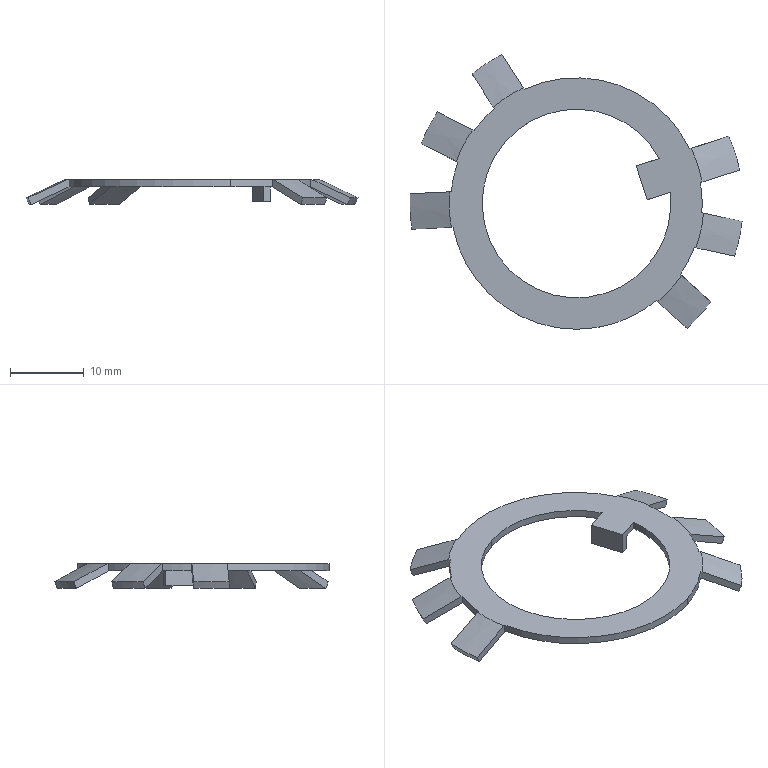Component | SolidWorks | 25RoundNutLockWasher(GB-T-858-1988)0-1 | 1 solid | 47 faces | box 44.9 x 37.13 x 3.38 mm | volume 592 mm3 | plane 19 | cone 18 | cylinder 10 | commonest cylinder face diameters 34 x7 25.5 x3 | material 45
build123d program:
from build123d import *

# Parameters (mm, degrees)
CUT_EXTRUDE1_DEPTH      = 10
CUT_EXTRUDE1_DEPTH_BACK = 10
SKETCH3_W               = 1
SKETCH3_H               = 4.8
BOSS_EXTRUDE1_DEPTH     = 2


with BuildPart() as part:
    # Sketch1 → Revolve1 (revolve)
    with BuildSketch(Plane.XY, mode=Mode.PRIVATE) as revolve1_sk:
        Polygon((0, 0.5), (0, -0.5), (17.222, -0.5), (22.516, 1.969), (22.093, 2.875), (17, 0.5), align=None)
    revolve(revolve1_sk.sketch.rotate(Axis((0, 2.914, 0), (0, -1, 0)), 90), axis=Axis((0, 2.914, 0), (0, -1, 0)))

    # Sketch2 → Cut-Extrude1 (cut, two sides: drawn at the far end of the back side and taken through both)
    with BuildSketch(Plane(origin=(0, 0.5, 0), x_dir=(1, 0, 0), z_dir=(0, 1, 0)).offset(-CUT_EXTRUDE1_DEPTH_BACK)):
        with BuildLine():
            Line((12.522, 2.4), (9.252, 2.4))
            Line((9.252, 2.4), (9.252, -2.4))
            Line((9.252, -2.4), (12.522, -2.4))
            ThreePointArc((12.522, -2.4), (-12.75, 0), (12.522, 2.4))
        make_face()
        with BuildLine():
            Line((16.83, 2.4), (25.795, 2.4))
            ThreePointArc((25.795, 2.4), (25.023, 6.705), (23.539, 10.819))
            Line((23.539, 10.819), (15.775, 6.336))
            ThreePointArc((15.775, 6.336), (16.421, 4.4), (16.83, 2.4))
        make_face()
        with BuildLine():
            Line((-16.542, -19.937), (-10.203, -13.597))
            ThreePointArc((-10.203, -13.597), (-8.5, -14.722), (-6.674, -15.635))
            Line((-6.674, -15.635), (-8.994, -24.295))
            ThreePointArc((-8.994, -24.295), (-12.953, -22.435), (-16.542, -19.937))
        make_face()
        with BuildLine():
            Line((25.795, -2.4), (16.83, -2.4))
            ThreePointArc((16.83, -2.4), (10.349, -13.487), (-2.038, -16.877))
            Line((-2.038, -16.877), (-4.358, -25.537))
            ThreePointArc((-4.358, -25.537), (15.771, -20.553), (25.795, -2.4))
        make_face()
        with BuildLine():
            Line((-13.597, -10.203), (-19.937, -16.542))
            ThreePointArc((-19.937, -16.542), (-22.435, -12.953), (-24.295, -8.994))
            Line((-24.295, -8.994), (-15.635, -6.674))
            ThreePointArc((-15.635, -6.674), (-14.722, -8.5), (-13.597, -10.203))
        make_face()
        with BuildLine():
            Line((13.375, 10.493), (21.139, 14.976))
            ThreePointArc((21.139, 14.976), (18.318, 18.318), (14.976, 21.139))
            Line((14.976, 21.139), (10.493, 13.375))
            ThreePointArc((10.493, 13.375), (12.021, 12.021), (13.375, 10.493))
        make_face()
        with BuildLine():
            Line((6.336, 15.775), (10.819, 23.539))
            ThreePointArc((10.819, 23.539), (-15.771, 20.553), (-25.537, -4.358))
            Line((-25.537, -4.358), (-16.877, -2.038))
            ThreePointArc((-16.877, -2.038), (-10.349, 13.487), (6.336, 15.775))
        make_face()
    extrude(amount=CUT_EXTRUDE1_DEPTH + CUT_EXTRUDE1_DEPTH_BACK, mode=Mode.SUBTRACT)

    # Sketch3 → Boss-Extrude1 (add)
    with BuildSketch(Plane(origin=(0, 0.5, 0), x_dir=(1, 0, 0), z_dir=(0, 1, 0))):
        with Locations((9.752, 0)):
            Rectangle(SKETCH3_W, SKETCH3_H)
    extrude(amount=BOSS_EXTRUDE1_DEPTH)


solid = part.part

# Placed as in the assembly
solid = solid.moved(Location((-15.093, -37.782, 204.755), (-90, -17.723, 0)))